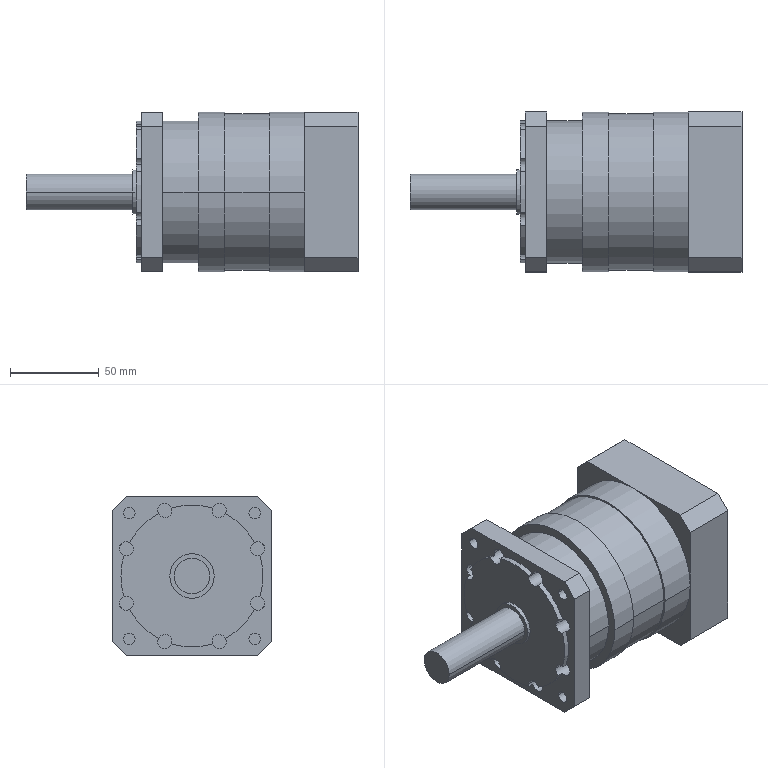Component | SolidWorks | MotorReducer-1 | 1 solid | 88 faces | box 187 x 90 x 90 mm | volume 816243 mm3 | cylinder 49 | plane 39 | commonest cylinder face diameters 8 x16 80 x13 6.5 x8 90 x4 22 x2 88 x2 20 x2 25 x2
build123d program:
from build123d import *

# Parameters (mm, degrees)
SKETCH2_W           = 90
SKETCH2_H           = 90
BOSS_EXTRUDE1_DEPTH = 30
CHAMFER1_SIZE       = 8
SKETCH9_R           = 45
BOSS_EXTRUDE3_DEPTH = 60
SKETCH11_R          = 40
BOSS_EXTRUDE5_DEPTH = 20
SKETCH12_W          = 90
SKETCH12_H          = 90
BOSS_EXTRUDE6_DEPTH = 12
CHAMFER3_SIZE       = 8
SKETCH13_R          = 40
BOSS_EXTRUDE7_DEPTH = 3
SKETCH14_R          = 12.5
BOSS_EXTRUDE8_DEPTH = 2
SKETCH15_R          = 10
BOSS_EXTRUDE9_DEPTH = 60
SKETCH16_W          = 1
SKETCH16_H          = 25
SKETCH18_R          = 3.25
CUT_EXTRUDE1_DEPTH  = 12
CIRPATTERN1_COUNT   = 4
SKETCH19_R          = 4
CUT_EXTRUDE2_DEPTH  = 10
CIRPATTERN2_COUNT   = 8
SKETCH20_R          = 40
CUT_EXTRUDE3_DEPTH  = 2
SKETCH21_R          = 11
CUT_EXTRUDE4_DEPTH  = 36


with BuildPart() as part:
    # Sketch2 → Boss-Extrude1 (new body)
    with BuildSketch(Plane.XY):
        Rectangle(SKETCH2_W, SKETCH2_H)
    extrude(amount=BOSS_EXTRUDE1_DEPTH)

    # Chamfer1
    chamfer1_edges = [part.edges().sort_by_distance(p)[0] for p in [
        (-45, 45, 15),
        (45, 45, 15),
        (45, -45, 15),
        (-45, -45, 15),
    ]]
    chamfer(chamfer1_edges, length=CHAMFER1_SIZE)

    # Sketch9 → Boss-Extrude3 (add)
    with BuildSketch(Plane.XY.offset(30)):
        Circle(SKETCH9_R)
    extrude(amount=BOSS_EXTRUDE3_DEPTH)

    # Sketch11 → Boss-Extrude5 (add)
    with BuildSketch(Plane.XY.offset(90)):
        Circle(SKETCH11_R)
    extrude(amount=BOSS_EXTRUDE5_DEPTH)

    # Sketch12 → Boss-Extrude6 (add)
    with BuildSketch(Plane.XY.offset(110)):
        Rectangle(SKETCH12_W, SKETCH12_H)
    extrude(amount=BOSS_EXTRUDE6_DEPTH)

    # Chamfer3
    chamfer3_edges = [part.edges().sort_by_distance(p)[0] for p in [
        (45, -45, 116),
        (45, 45, 116),
        (-45, 45, 116),
        (-45, -45, 116),
    ]]
    chamfer(chamfer3_edges, length=CHAMFER3_SIZE)

    # Sketch13 → Boss-Extrude7 (add)
    with BuildSketch(Plane.XY.offset(122)):
        Circle(SKETCH13_R)
    extrude(amount=BOSS_EXTRUDE7_DEPTH)

    # Sketch14 → Boss-Extrude8 (add)
    with BuildSketch(Plane.XY.offset(125)):
        Circle(SKETCH14_R)
    extrude(amount=BOSS_EXTRUDE8_DEPTH)

    # Sketch15 → Boss-Extrude9 (add)
    with BuildSketch(Plane.XY.offset(127)):
        Circle(SKETCH15_R)
    extrude(amount=BOSS_EXTRUDE9_DEPTH)

    # Cut-Sweep1: sweep along a path in Sketch17
    with BuildLine(Plane.XY.offset(75)) as cut_sweep1_path:
        CenterArc((0, 0), 45, 0, 360)
    # Sketch16 → Cut-Sweep1 (sweep, cut)
    with BuildSketch(Plane(origin=(0, 0, 0), x_dir=(1, 0, 0), z_dir=(0, 1, 0))):
        with Locations((-44.5, -62.5)):
            Rectangle(SKETCH16_W, SKETCH16_H)
    sweep(path=cut_sweep1_path.line, mode=Mode.SUBTRACT)

    # Sketch18 → Cut-Extrude1 (cut)
    with BuildSketch(Plane.XY.offset(122)):
        with Locations((-35.355, 35.355)):
            Circle(SKETCH18_R)
    cut_extrude1 = extrude(amount=-CUT_EXTRUDE1_DEPTH, mode=Mode.SUBTRACT)

    # CirPattern1: Cut-Extrude1 ×4 about axis
    cirpattern1_axis = Axis((0, 0, 0), (0, 0, 1))
    for i in range(1, CIRPATTERN1_COUNT):
        add(cut_extrude1.rotate(cirpattern1_axis, i * 360 / CIRPATTERN1_COUNT), mode=Mode.SUBTRACT)

    # Sketch19 → Cut-Extrude2 (cut)
    with BuildSketch(Plane.XY.offset(125)):
        with Locations((15.307, 36.955)):
            Circle(SKETCH19_R)
    cut_extrude2 = extrude(amount=-CUT_EXTRUDE2_DEPTH, mode=Mode.SUBTRACT)

    # CirPattern2: Cut-Extrude2 ×8 about axis
    cirpattern2_axis = Axis((0, 0, 0), (0, 0, 1))
    for i in range(1, CIRPATTERN2_COUNT):
        add(cut_extrude2.rotate(cirpattern2_axis, i * 360 / CIRPATTERN2_COUNT), mode=Mode.SUBTRACT)

    # Sketch20 → Cut-Extrude3 (cut)
    with BuildSketch(Plane(origin=(0, 0, 0), x_dir=(-1, 0, 0), z_dir=(0, 0, -1))):
        with Locations(Location((0, 0, 0), (0, 0, 180))):
            Circle(SKETCH20_R)
    extrude(amount=-CUT_EXTRUDE3_DEPTH, mode=Mode.SUBTRACT)

    # Sketch21 → Cut-Extrude4 (cut)
    with BuildSketch(Plane(origin=(0, 0, 2), x_dir=(-1, 0, 0), z_dir=(0, 0, -1))):
        Circle(SKETCH21_R)
    extrude(amount=-CUT_EXTRUDE4_DEPTH, mode=Mode.SUBTRACT)


solid = part.part

# Placed as in the assembly
solid = solid.moved(Location((-432.371, -1090.9, 148), (0, -90, 0)))